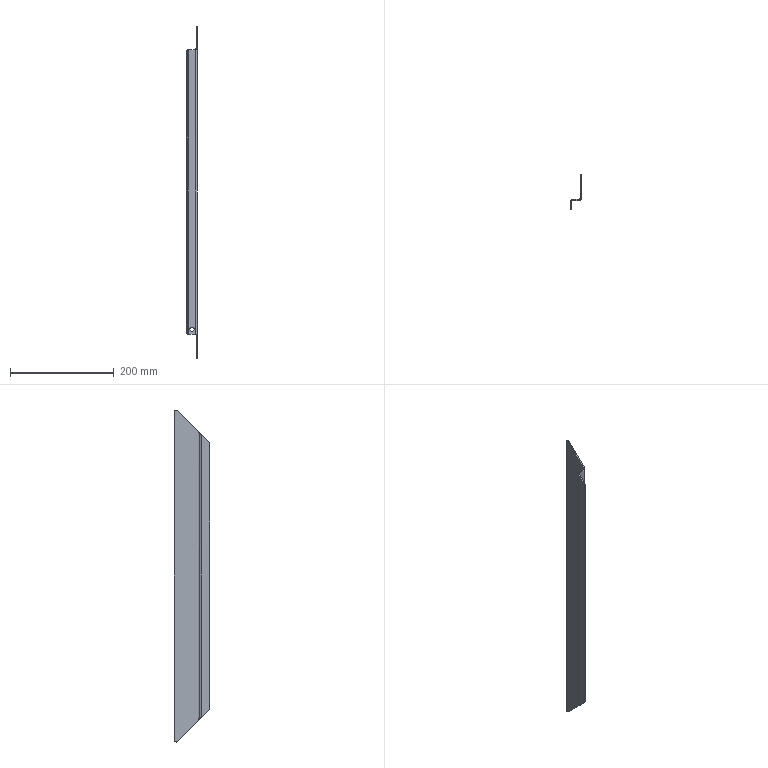Component | SolidWorks | BoxWelding-1_FrontAndRearPlate3-1 | 1 solid | 27 faces | box 20 x 68 x 641.51 mm | volume 95964 mm3 | plane 14 | cylinder 9 | spline 4 | commonest cylinder face diameters 8 x4 6 x3 4 x2
STEP:
#1=COLOUR_RGB('',0.7922,0.8196,0.9333);
#2=FILL_AREA_STYLE_COLOUR('',#1);
#3=FILL_AREA_STYLE('',(#2));
#4=SURFACE_STYLE_FILL_AREA(#3);
#5=SURFACE_SIDE_STYLE('',(#4));
#6=SURFACE_STYLE_USAGE(.BOTH.,#5);
#7=PRESENTATION_STYLE_ASSIGNMENT((#6));
#8=CARTESIAN_POINT('',(22.269,49.429,-6.496));
#9=VERTEX_POINT('',#8);
#10=CARTESIAN_POINT('',(21.954,49.429,-6.496));
#11=VERTEX_POINT('',#10);
#12=CARTESIAN_POINT('',(22.111,49.429,-6.496));
#13=DIRECTION('',(0.,-1.,0.));
#14=DIRECTION('',(-1.,0.,-0.));
#15=AXIS2_PLACEMENT_3D('',#12,#13,#14);
#16=CIRCLE('',#15,0.1575);
#17=EDGE_CURVE('',#9,#11,#16,.T.);
#18=ORIENTED_EDGE('',*,*,#17,.F.);
#19=CARTESIAN_POINT('',(22.269,49.35,-6.496));
#20=VERTEX_POINT('',#19);
#21=CARTESIAN_POINT('',(22.269,49.744,-6.496));
#22=DIRECTION('',(0.,-1.,0.));
#23=VECTOR('',#22,39.37);
#24=LINE('',#21,#23);
#25=EDGE_CURVE('',#9,#20,#24,.T.);
#26=ORIENTED_EDGE('',*,*,#25,.T.);
#27=CARTESIAN_POINT('',(21.954,49.35,-6.496));
#28=VERTEX_POINT('',#27);
#29=CARTESIAN_POINT('',(22.111,49.35,-6.496));
#30=DIRECTION('',(0.,-1.,0.));
#31=DIRECTION('',(-1.,0.,-0.));
#32=AXIS2_PLACEMENT_3D('',#29,#30,#31);
#33=CIRCLE('',#32,0.1575);
#34=EDGE_CURVE('',#20,#28,#33,.T.);
#35=ORIENTED_EDGE('',*,*,#34,.T.);
#36=CARTESIAN_POINT('',(21.954,49.744,-6.496));
#37=DIRECTION('',(0.,-1.,0.));
#38=VECTOR('',#37,39.37);
#39=LINE('',#36,#38);
#40=EDGE_CURVE('',#11,#28,#39,.T.);
#41=ORIENTED_EDGE('',*,*,#40,.F.);
#42=EDGE_LOOP('',(#18,#26,#35,#41));
#43=FACE_OUTER_BOUND('',#42,.T.);
#44=CARTESIAN_POINT('',(22.111,49.744,-6.496));
#45=DIRECTION('',(0.,-1.,0.));
#46=DIRECTION('',(-1.,0.,-0.));
#47=AXIS2_PLACEMENT_3D('',#44,#45,#46);
#48=CYLINDRICAL_SURFACE('',#47,0.1575);
#49=ADVANCED_FACE('',(#43),#48,.F.);
#50=CARTESIAN_POINT('',(22.505,51.201,16.566));
#51=VERTEX_POINT('',#50);
#52=CARTESIAN_POINT('',(22.505,51.117,16.531));
#53=VERTEX_POINT('',#52);
#54=CARTESIAN_POINT('',(22.505,51.201,16.448));
#55=DIRECTION('',(1.,0.,0.));
#56=DIRECTION('',(0.,-0.,-1.));
#57=AXIS2_PLACEMENT_3D('',#54,#55,#56);
#58=CIRCLE('',#57,0.1181);
#59=EDGE_CURVE('',#51,#53,#58,.T.);
#60=ORIENTED_EDGE('',*,*,#59,.F.);
#61=CARTESIAN_POINT('',(22.426,51.201,16.566));
#62=VERTEX_POINT('',#61);
#63=CARTESIAN_POINT('',(22.505,51.201,16.566));
#64=DIRECTION('',(-1.,-0.,-0.));
#65=VECTOR('',#64,39.37);
#66=LINE('',#63,#65);
#67=EDGE_CURVE('',#51,#62,#66,.T.);
#68=ORIENTED_EDGE('',*,*,#67,.T.);
#69=CARTESIAN_POINT('',(22.426,51.117,16.531));
#70=VERTEX_POINT('',#69);
#71=CARTESIAN_POINT('',(22.426,51.201,16.448));
#72=DIRECTION('',(-1.,-0.,-0.));
#73=DIRECTION('',(0.,-0.,-1.));
#74=AXIS2_PLACEMENT_3D('',#71,#72,#73);
#75=CIRCLE('',#74,0.1181);
#76=EDGE_CURVE('',#70,#62,#75,.T.);
#77=ORIENTED_EDGE('',*,*,#76,.F.);
#78=CARTESIAN_POINT('',(22.426,51.117,16.531));
#79=DIRECTION('',(-1.,-0.,-0.));
#80=VECTOR('',#79,39.37);
#81=LINE('',#78,#80);
#82=EDGE_CURVE('',#53,#70,#81,.T.);
#83=ORIENTED_EDGE('',*,*,#82,.F.);
#84=EDGE_LOOP('',(#60,#68,#77,#83));
#85=FACE_OUTER_BOUND('',#84,.T.);
#86=CARTESIAN_POINT('',(22.505,51.201,16.448));
#87=DIRECTION('',(-1.,-0.,-0.));
#88=DIRECTION('',(0.,0.,1.));
#89=AXIS2_PLACEMENT_3D('',#86,#87,#88);
#90=CYLINDRICAL_SURFACE('',#89,0.1181);
#91=ADVANCED_FACE('',(#85),#90,.T.);
#92=CARTESIAN_POINT('',(22.111,49.35,-6.496));
#93=DIRECTION('',(0.,-1.,0.));
#94=DIRECTION('',(-1.,0.,-0.));
#95=AXIS2_PLACEMENT_3D('',#92,#93,#94);
#96=CIRCLE('',#95,0.1575);
#97=EDGE_CURVE('',#28,#20,#96,.T.);
#98=ORIENTED_EDGE('',*,*,#97,.F.);
#99=ORIENTED_EDGE('',*,*,#34,.F.);
#100=EDGE_LOOP('',(#98,#99));
#101=FACE_BOUND('',#100,.T.);
#102=CARTESIAN_POINT('',(22.347,49.35,-6.889));
#103=VERTEX_POINT('',#102);
#104=CARTESIAN_POINT('',(22.347,49.35,14.764));
#105=VERTEX_POINT('',#104);
#106=CARTESIAN_POINT('',(22.347,49.35,16.733));
#107=DIRECTION('',(-0.,0.,1.));
#108=VECTOR('',#107,39.37);
#109=LINE('',#106,#108);
#110=EDGE_CURVE('',#103,#105,#109,.T.);
#111=ORIENTED_EDGE('',*,*,#110,.T.);
#112=CARTESIAN_POINT('',(21.875,49.35,14.764));
#113=VERTEX_POINT('',#112);
#114=CARTESIAN_POINT('',(22.426,49.35,14.764));
#115=DIRECTION('',(1.,0.,0.));
#116=VECTOR('',#115,39.37);
#117=LINE('',#114,#116);
#118=EDGE_CURVE('',#113,#105,#117,.T.);
#119=ORIENTED_EDGE('',*,*,#118,.F.);
#120=CARTESIAN_POINT('',(21.875,49.35,-6.889));
#121=VERTEX_POINT('',#120);
#122=CARTESIAN_POINT('',(21.875,49.35,-8.858));
#123=DIRECTION('',(-0.,0.,1.));
#124=VECTOR('',#123,39.37);
#125=LINE('',#122,#124);
#126=EDGE_CURVE('',#121,#113,#125,.T.);
#127=ORIENTED_EDGE('',*,*,#126,.F.);
#128=CARTESIAN_POINT('',(22.426,49.35,-6.889));
#129=DIRECTION('',(-1.,-0.,-0.));
#130=VECTOR('',#129,39.37);
#131=LINE('',#128,#130);
#132=EDGE_CURVE('',#103,#121,#131,.T.);
#133=ORIENTED_EDGE('',*,*,#132,.F.);
#134=EDGE_LOOP('',(#111,#119,#127,#133));
#135=FACE_OUTER_BOUND('',#134,.T.);
#136=CARTESIAN_POINT('',(22.426,49.35,16.733));
#137=DIRECTION('',(0.,-1.,0.));
#138=DIRECTION('',(-1.,-0.,-0.));
#139=AXIS2_PLACEMENT_3D('',#136,#137,#138);
#140=PLANE('',#139);
#141=ADVANCED_FACE('',(#101,#135),#140,.T.);
#142=CARTESIAN_POINT('',(22.111,49.429,-6.496));
#143=DIRECTION('',(0.,-1.,0.));
#144=DIRECTION('',(-1.,0.,-0.));
#145=AXIS2_PLACEMENT_3D('',#142,#143,#144);
#146=CIRCLE('',#145,0.1575);
#147=EDGE_CURVE('',#11,#9,#146,.T.);
#148=ORIENTED_EDGE('',*,*,#147,.T.);
#149=ORIENTED_EDGE('',*,*,#17,.T.);
#150=EDGE_LOOP('',(#148,#149));
#151=FACE_BOUND('',#150,.T.);
#152=CARTESIAN_POINT('',(21.875,49.429,14.764));
#153=VERTEX_POINT('',#152);
#154=CARTESIAN_POINT('',(22.347,49.429,14.764));
#155=VERTEX_POINT('',#154);
#156=CARTESIAN_POINT('',(22.426,49.429,14.764));
#157=DIRECTION('',(1.,0.,0.));
#158=VECTOR('',#157,39.37);
#159=LINE('',#156,#158);
#160=EDGE_CURVE('',#153,#155,#159,.T.);
#161=ORIENTED_EDGE('',*,*,#160,.T.);
#162=CARTESIAN_POINT('',(22.347,49.429,-6.889));
#163=VERTEX_POINT('',#162);
#164=CARTESIAN_POINT('',(22.347,49.429,-8.858));
#165=DIRECTION('',(-0.,0.,1.));
#166=VECTOR('',#165,39.37);
#167=LINE('',#164,#166);
#168=EDGE_CURVE('',#163,#155,#167,.T.);
#169=ORIENTED_EDGE('',*,*,#168,.F.);
#170=CARTESIAN_POINT('',(21.875,49.429,-6.889));
#171=VERTEX_POINT('',#170);
#172=CARTESIAN_POINT('',(22.426,49.429,-6.889));
#173=DIRECTION('',(-1.,-0.,-0.));
#174=VECTOR('',#173,39.37);
#175=LINE('',#172,#174);
#176=EDGE_CURVE('',#163,#171,#175,.T.);
#177=ORIENTED_EDGE('',*,*,#176,.T.);
#178=CARTESIAN_POINT('',(21.875,49.429,-8.858));
#179=DIRECTION('',(-0.,0.,1.));
#180=VECTOR('',#179,39.37);
#181=LINE('',#178,#180);
#182=EDGE_CURVE('',#171,#153,#181,.T.);
#183=ORIENTED_EDGE('',*,*,#182,.T.);
#184=EDGE_LOOP('',(#161,#169,#177,#183));
#185=FACE_OUTER_BOUND('',#184,.T.);
#186=CARTESIAN_POINT('',(22.426,49.429,16.733));
#187=DIRECTION('',(0.,-1.,0.));
#188=DIRECTION('',(-1.,-0.,-0.));
#189=AXIS2_PLACEMENT_3D('',#186,#187,#188);
#190=PLANE('',#189);
#191=ADVANCED_FACE('',(#151,#185),#190,.F.);
#192=CARTESIAN_POINT('',(22.505,51.319,-8.573));
#193=VERTEX_POINT('',#192);
#194=CARTESIAN_POINT('',(22.505,51.319,16.448));
#195=VERTEX_POINT('',#194);
#196=CARTESIAN_POINT('',(22.505,51.319,16.733));
#197=DIRECTION('',(-0.,0.,1.));
#198=VECTOR('',#197,39.37);
#199=LINE('',#196,#198);
#200=EDGE_CURVE('',#193,#195,#199,.T.);
#201=ORIENTED_EDGE('',*,*,#200,.T.);
#202=CARTESIAN_POINT('',(22.505,51.201,16.448));
#203=DIRECTION('',(1.,0.,0.));
#204=DIRECTION('',(0.,-0.,-1.));
#205=AXIS2_PLACEMENT_3D('',#202,#203,#204);
#206=CIRCLE('',#205,0.1181);
#207=EDGE_CURVE('',#195,#51,#206,.T.);
#208=ORIENTED_EDGE('',*,*,#207,.T.);
#209=ORIENTED_EDGE('',*,*,#59,.T.);
#210=CARTESIAN_POINT('',(22.505,49.508,14.922));
#211=VERTEX_POINT('',#210);
#212=CARTESIAN_POINT('',(22.505,37.539,2.953));
#213=DIRECTION('',(-0.,0.7071,0.7071));
#214=VECTOR('',#213,39.37);
#215=LINE('',#212,#214);
#216=EDGE_CURVE('',#211,#53,#215,.T.);
#217=ORIENTED_EDGE('',*,*,#216,.F.);
#218=CARTESIAN_POINT('',(22.505,49.508,-7.047));
#219=VERTEX_POINT('',#218);
#220=CARTESIAN_POINT('',(22.505,49.508,16.733));
#221=DIRECTION('',(0.,-0.,-1.));
#222=VECTOR('',#221,39.37);
#223=LINE('',#220,#222);
#224=EDGE_CURVE('',#211,#219,#223,.T.);
#225=ORIENTED_EDGE('',*,*,#224,.T.);
#226=CARTESIAN_POINT('',(22.505,51.117,-8.656));
#227=VERTEX_POINT('',#226);
#228=CARTESIAN_POINT('',(22.505,50.335,-7.874));
#229=DIRECTION('',(0.,-0.7071,0.7071));
#230=VECTOR('',#229,39.37);
#231=LINE('',#228,#230);
#232=EDGE_CURVE('',#227,#219,#231,.T.);
#233=ORIENTED_EDGE('',*,*,#232,.F.);
#234=CARTESIAN_POINT('',(22.505,51.201,-8.573));
#235=DIRECTION('',(1.,0.,0.));
#236=DIRECTION('',(0.,-0.,-1.));
#237=AXIS2_PLACEMENT_3D('',#234,#235,#236);
#238=CIRCLE('',#237,0.1181);
#239=EDGE_CURVE('',#227,#193,#238,.T.);
#240=ORIENTED_EDGE('',*,*,#239,.T.);
#241=EDGE_LOOP('',(#201,#208,#209,#217,#225,#233,#240));
#242=FACE_OUTER_BOUND('',#241,.T.);
#243=CARTESIAN_POINT('',(22.505,49.35,-8.858));
#244=DIRECTION('',(1.,0.,0.));
#245=DIRECTION('',(0.,-0.,-1.));
#246=AXIS2_PLACEMENT_3D('',#243,#244,#245);
#247=PLANE('',#246);
#248=ADVANCED_FACE('',(#242),#247,.T.);
#249=CARTESIAN_POINT('',(22.426,49.508,14.922));
#250=VERTEX_POINT('',#249);
#251=CARTESIAN_POINT('',(22.426,37.539,2.953));
#252=DIRECTION('',(-0.,0.7071,0.7071));
#253=VECTOR('',#252,39.37);
#254=LINE('',#251,#253);
#255=EDGE_CURVE('',#250,#70,#254,.T.);
#256=ORIENTED_EDGE('',*,*,#255,.T.);
#257=ORIENTED_EDGE('',*,*,#76,.T.);
#258=CARTESIAN_POINT('',(22.426,51.319,16.448));
#259=VERTEX_POINT('',#258);
#260=CARTESIAN_POINT('',(22.426,51.201,16.448));
#261=DIRECTION('',(-1.,-0.,-0.));
#262=DIRECTION('',(0.,-0.,-1.));
#263=AXIS2_PLACEMENT_3D('',#260,#261,#262);
#264=CIRCLE('',#263,0.1181);
#265=EDGE_CURVE('',#62,#259,#264,.T.);
#266=ORIENTED_EDGE('',*,*,#265,.T.);
#267=CARTESIAN_POINT('',(22.426,51.319,-8.573));
#268=VERTEX_POINT('',#267);
#269=CARTESIAN_POINT('',(22.426,51.319,-8.858));
#270=DIRECTION('',(-0.,0.,1.));
#271=VECTOR('',#270,39.37);
#272=LINE('',#269,#271);
#273=EDGE_CURVE('',#268,#259,#272,.T.);
#274=ORIENTED_EDGE('',*,*,#273,.F.);
#275=CARTESIAN_POINT('',(22.426,51.117,-8.656));
#276=VERTEX_POINT('',#275);
#277=CARTESIAN_POINT('',(22.426,51.201,-8.573));
#278=DIRECTION('',(-1.,-0.,-0.));
#279=DIRECTION('',(0.,-0.,-1.));
#280=AXIS2_PLACEMENT_3D('',#277,#278,#279);
#281=CIRCLE('',#280,0.1181);
#282=EDGE_CURVE('',#268,#276,#281,.T.);
#283=ORIENTED_EDGE('',*,*,#282,.T.);
#284=CARTESIAN_POINT('',(22.426,49.508,-7.047));
#285=VERTEX_POINT('',#284);
#286=CARTESIAN_POINT('',(22.426,50.335,-7.874));
#287=DIRECTION('',(0.,-0.7071,0.7071));
#288=VECTOR('',#287,39.37);
#289=LINE('',#286,#288);
#290=EDGE_CURVE('',#276,#285,#289,.T.);
#291=ORIENTED_EDGE('',*,*,#290,.T.);
#292=CARTESIAN_POINT('',(22.426,49.508,16.733));
#293=DIRECTION('',(0.,-0.,-1.));
#294=VECTOR('',#293,39.37);
#295=LINE('',#292,#294);
#296=EDGE_CURVE('',#250,#285,#295,.T.);
#297=ORIENTED_EDGE('',*,*,#296,.F.);
#298=EDGE_LOOP('',(#256,#257,#266,#274,#283,#291,#297));
#299=FACE_OUTER_BOUND('',#298,.T.);
#300=CARTESIAN_POINT('',(22.426,49.35,-8.858));
#301=DIRECTION('',(1.,0.,0.));
#302=DIRECTION('',(0.,-0.,-1.));
#303=AXIS2_PLACEMENT_3D('',#300,#301,#302);
#304=PLANE('',#303);
#305=ADVANCED_FACE('',(#299),#304,.F.);
#306=ORIENTED_EDGE('',*,*,#224,.F.);
#307=CARTESIAN_POINT('',(22.347,49.35,14.764));
#308=CARTESIAN_POINT('',(22.44,49.35,14.764));
#309=CARTESIAN_POINT('',(22.505,49.416,14.83));
#310=CARTESIAN_POINT('',(22.505,49.508,14.922));
#311=(BOUNDED_CURVE()B_SPLINE_CURVE(3,(#307,#308,#309,#310),.UNSPECIFIED.,.F.,.T.)B_SPLINE_CURVE_WITH_KNOTS((4,4),(3.142,4.712),.UNSPECIFIED.)CURVE()GEOMETRIC_REPRESENTATION_ITEM()RATIONAL_B_SPLINE_CURVE((1.,0.8047,0.8047,1.))REPRESENTATION_ITEM(''));
#312=EDGE_CURVE('',#105,#211,#311,.T.);
#313=ORIENTED_EDGE('',*,*,#312,.F.);
#314=ORIENTED_EDGE('',*,*,#110,.F.);
#315=CARTESIAN_POINT('',(22.505,49.508,-7.047));
#316=CARTESIAN_POINT('',(22.505,49.416,-6.954));
#317=CARTESIAN_POINT('',(22.44,49.35,-6.889));
#318=CARTESIAN_POINT('',(22.347,49.35,-6.889));
#319=(BOUNDED_CURVE()B_SPLINE_CURVE(3,(#315,#316,#317,#318),.UNSPECIFIED.,.F.,.F.)B_SPLINE_CURVE_WITH_KNOTS((4,4),(4.712,6.283),.UNSPECIFIED.)CURVE()GEOMETRIC_REPRESENTATION_ITEM()RATIONAL_B_SPLINE_CURVE((1.,0.8047,0.8047,1.))REPRESENTATION_ITEM(''));
#320=EDGE_CURVE('',#219,#103,#319,.T.);
#321=ORIENTED_EDGE('',*,*,#320,.F.);
#322=EDGE_LOOP('',(#306,#313,#314,#321));
#323=FACE_OUTER_BOUND('',#322,.T.);
#324=CARTESIAN_POINT('',(22.347,49.508,16.733));
#325=DIRECTION('',(-0.,0.,1.));
#326=DIRECTION('',(0.,-1.,0.));
#327=AXIS2_PLACEMENT_3D('',#324,#325,#326);
#328=CYLINDRICAL_SURFACE('',#327,0.1575);
#329=ADVANCED_FACE('',(#323),#328,.T.);
#330=CARTESIAN_POINT('',(22.347,49.429,14.764));
#331=CARTESIAN_POINT('',(22.393,49.429,14.764));
#332=CARTESIAN_POINT('',(22.426,49.462,14.83));
#333=CARTESIAN_POINT('',(22.426,49.508,14.922));
#334=(BOUNDED_CURVE()B_SPLINE_CURVE(3,(#330,#331,#332,#333),.UNSPECIFIED.,.F.,.F.)B_SPLINE_CURVE_WITH_KNOTS((4,4),(3.142,4.712),.UNSPECIFIED.)CURVE()GEOMETRIC_REPRESENTATION_ITEM()RATIONAL_B_SPLINE_CURVE((1.,0.8047,0.8047,1.))REPRESENTATION_ITEM(''));
#335=EDGE_CURVE('',#155,#250,#334,.T.);
#336=ORIENTED_EDGE('',*,*,#335,.T.);
#337=ORIENTED_EDGE('',*,*,#296,.T.);
#338=CARTESIAN_POINT('',(22.426,49.508,-7.047));
#339=CARTESIAN_POINT('',(22.426,49.462,-6.954));
#340=CARTESIAN_POINT('',(22.393,49.429,-6.889));
#341=CARTESIAN_POINT('',(22.347,49.429,-6.889));
#342=(BOUNDED_CURVE()B_SPLINE_CURVE(3,(#338,#339,#340,#341),.UNSPECIFIED.,.F.,.F.)B_SPLINE_CURVE_WITH_KNOTS((4,4),(4.712,6.283),.UNSPECIFIED.)CURVE()GEOMETRIC_REPRESENTATION_ITEM()RATIONAL_B_SPLINE_CURVE((1.,0.8047,0.8047,1.))REPRESENTATION_ITEM(''));
#343=EDGE_CURVE('',#285,#163,#342,.T.);
#344=ORIENTED_EDGE('',*,*,#343,.T.);
#345=ORIENTED_EDGE('',*,*,#168,.T.);
#346=EDGE_LOOP('',(#336,#337,#344,#345));
#347=FACE_OUTER_BOUND('',#346,.T.);
#348=CARTESIAN_POINT('',(22.347,49.508,16.733));
#349=DIRECTION('',(-0.,0.,1.));
#350=DIRECTION('',(0.,-1.,0.));
#351=AXIS2_PLACEMENT_3D('',#348,#349,#350);
#352=CYLINDRICAL_SURFACE('',#351,0.07874);
#353=ADVANCED_FACE('',(#347),#352,.F.);
#354=CARTESIAN_POINT('',(21.717,49.272,14.686));
#355=VERTEX_POINT('',#354);
#356=CARTESIAN_POINT('',(21.717,49.272,-6.811));
#357=VERTEX_POINT('',#356);
#358=CARTESIAN_POINT('',(21.717,49.272,-8.858));
#359=DIRECTION('',(0.,-0.,-1.));
#360=VECTOR('',#359,39.37);
#361=LINE('',#358,#360);
#362=EDGE_CURVE('',#355,#357,#361,.T.);
#363=ORIENTED_EDGE('',*,*,#362,.F.);
#364=CARTESIAN_POINT('',(21.875,49.429,14.764));
#365=CARTESIAN_POINT('',(21.783,49.429,14.764));
#366=CARTESIAN_POINT('',(21.717,49.364,14.732));
#367=CARTESIAN_POINT('',(21.717,49.272,14.686));
#368=(BOUNDED_CURVE()B_SPLINE_CURVE(3,(#364,#365,#366,#367),.UNSPECIFIED.,.F.,.T.)B_SPLINE_CURVE_WITH_KNOTS((4,4),(3.142,4.712),.UNSPECIFIED.)CURVE()GEOMETRIC_REPRESENTATION_ITEM()RATIONAL_B_SPLINE_CURVE((1.,0.8047,0.8047,1.))REPRESENTATION_ITEM(''));
#369=EDGE_CURVE('',#153,#355,#368,.T.);
#370=ORIENTED_EDGE('',*,*,#369,.F.);
#371=ORIENTED_EDGE('',*,*,#182,.F.);
#372=CARTESIAN_POINT('',(21.717,49.272,-6.811));
#373=CARTESIAN_POINT('',(21.717,49.364,-6.857));
#374=CARTESIAN_POINT('',(21.783,49.429,-6.889));
#375=CARTESIAN_POINT('',(21.875,49.429,-6.889));
#376=(BOUNDED_CURVE()B_SPLINE_CURVE(3,(#372,#373,#374,#375),.UNSPECIFIED.,.F.,.T.)B_SPLINE_CURVE_WITH_KNOTS((4,4),(4.712,6.283),.UNSPECIFIED.)CURVE()GEOMETRIC_REPRESENTATION_ITEM()RATIONAL_B_SPLINE_CURVE((1.,0.8047,0.8047,1.))REPRESENTATION_ITEM(''));
#377=EDGE_CURVE('',#357,#171,#376,.T.);
#378=ORIENTED_EDGE('',*,*,#377,.F.);
#379=EDGE_LOOP('',(#363,#370,#371,#378));
#380=FACE_OUTER_BOUND('',#379,.T.);
#381=CARTESIAN_POINT('',(21.875,49.272,-8.858));
#382=DIRECTION('',(0.,-0.,-1.));
#383=DIRECTION('',(-1.,0.,-0.));
#384=AXIS2_PLACEMENT_3D('',#381,#382,#383);
#385=CYLINDRICAL_SURFACE('',#384,0.1575);
#386=ADVANCED_FACE('',(#380),#385,.T.);
#387=CARTESIAN_POINT('',(21.796,49.272,14.686));
#388=VERTEX_POINT('',#387);
#389=CARTESIAN_POINT('',(21.875,49.35,14.764));
#390=CARTESIAN_POINT('',(21.829,49.35,14.764));
#391=CARTESIAN_POINT('',(21.796,49.318,14.732));
#392=CARTESIAN_POINT('',(21.796,49.272,14.686));
#393=(BOUNDED_CURVE()B_SPLINE_CURVE(3,(#389,#390,#391,#392),.UNSPECIFIED.,.F.,.F.)B_SPLINE_CURVE_WITH_KNOTS((4,4),(3.142,4.712),.UNSPECIFIED.)CURVE()GEOMETRIC_REPRESENTATION_ITEM()RATIONAL_B_SPLINE_CURVE((1.,0.8047,0.8047,1.))REPRESENTATION_ITEM(''));
#394=EDGE_CURVE('',#113,#388,#393,.T.);
#395=ORIENTED_EDGE('',*,*,#394,.T.);
#396=CARTESIAN_POINT('',(21.796,49.272,-6.811));
#397=VERTEX_POINT('',#396);
#398=CARTESIAN_POINT('',(21.796,49.272,16.733));
#399=DIRECTION('',(0.,-0.,-1.));
#400=VECTOR('',#399,39.37);
#401=LINE('',#398,#400);
#402=EDGE_CURVE('',#388,#397,#401,.T.);
#403=ORIENTED_EDGE('',*,*,#402,.T.);
#404=CARTESIAN_POINT('',(21.796,49.272,-6.811));
#405=CARTESIAN_POINT('',(21.796,49.318,-6.857));
#406=CARTESIAN_POINT('',(21.829,49.35,-6.889));
#407=CARTESIAN_POINT('',(21.875,49.35,-6.889));
#408=(BOUNDED_CURVE()B_SPLINE_CURVE(3,(#404,#405,#406,#407),.UNSPECIFIED.,.F.,.F.)B_SPLINE_CURVE_WITH_KNOTS((4,4),(4.712,6.283),.UNSPECIFIED.)CURVE()GEOMETRIC_REPRESENTATION_ITEM()RATIONAL_B_SPLINE_CURVE((1.,0.8047,0.8047,1.))REPRESENTATION_ITEM(''));
#409=EDGE_CURVE('',#397,#121,#408,.T.);
#410=ORIENTED_EDGE('',*,*,#409,.T.);
#411=ORIENTED_EDGE('',*,*,#126,.T.);
#412=EDGE_LOOP('',(#395,#403,#410,#411));
#413=FACE_OUTER_BOUND('',#412,.T.);
#414=CARTESIAN_POINT('',(21.875,49.272,-8.858));
#415=DIRECTION('',(0.,-0.,-1.));
#416=DIRECTION('',(-1.,0.,0.));
#417=AXIS2_PLACEMENT_3D('',#414,#415,#416);
#418=CYLINDRICAL_SURFACE('',#417,0.07874);
#419=ADVANCED_FACE('',(#413),#418,.F.);
#420=CARTESIAN_POINT('',(21.717,48.642,14.056));
#421=VERTEX_POINT('',#420);
#422=CARTESIAN_POINT('',(21.717,48.642,-6.181));
#423=VERTEX_POINT('',#422);
#424=CARTESIAN_POINT('',(21.717,48.642,-8.858));
#425=DIRECTION('',(0.,-0.,-1.));
#426=VECTOR('',#425,39.37);
#427=LINE('',#424,#426);
#428=EDGE_CURVE('',#421,#423,#427,.T.);
#429=ORIENTED_EDGE('',*,*,#428,.F.);
#430=CARTESIAN_POINT('',(21.717,37.539,2.953));
#431=DIRECTION('',(0.,-0.7071,-0.7071));
#432=VECTOR('',#431,39.37);
#433=LINE('',#430,#432);
#434=EDGE_CURVE('',#355,#421,#433,.T.);
#435=ORIENTED_EDGE('',*,*,#434,.F.);
#436=ORIENTED_EDGE('',*,*,#362,.T.);
#437=CARTESIAN_POINT('',(21.717,51.319,-8.858));
#438=DIRECTION('',(0.,-0.7071,0.7071));
#439=VECTOR('',#438,39.37);
#440=LINE('',#437,#439);
#441=EDGE_CURVE('',#357,#423,#440,.T.);
#442=ORIENTED_EDGE('',*,*,#441,.T.);
#443=EDGE_LOOP('',(#429,#435,#436,#442));
#444=FACE_OUTER_BOUND('',#443,.T.);
#445=CARTESIAN_POINT('',(21.717,49.35,-8.858));
#446=DIRECTION('',(-1.,-0.,-0.));
#447=DIRECTION('',(-0.,0.,1.));
#448=AXIS2_PLACEMENT_3D('',#445,#446,#447);
#449=PLANE('',#448);
#450=ADVANCED_FACE('',(#444),#449,.T.);
#451=CARTESIAN_POINT('',(21.796,48.642,14.056));
#452=VERTEX_POINT('',#451);
#453=CARTESIAN_POINT('',(21.796,37.539,2.953));
#454=DIRECTION('',(0.,-0.7071,-0.7071));
#455=VECTOR('',#454,39.37);
#456=LINE('',#453,#455);
#457=EDGE_CURVE('',#388,#452,#456,.T.);
#458=ORIENTED_EDGE('',*,*,#457,.T.);
#459=CARTESIAN_POINT('',(21.796,48.642,-6.181));
#460=VERTEX_POINT('',#459);
#461=CARTESIAN_POINT('',(21.796,48.642,-8.858));
#462=DIRECTION('',(0.,-0.,-1.));
#463=VECTOR('',#462,39.37);
#464=LINE('',#461,#463);
#465=EDGE_CURVE('',#452,#460,#464,.T.);
#466=ORIENTED_EDGE('',*,*,#465,.T.);
#467=CARTESIAN_POINT('',(21.796,51.319,-8.858));
#468=DIRECTION('',(0.,-0.7071,0.7071));
#469=VECTOR('',#468,39.37);
#470=LINE('',#467,#469);
#471=EDGE_CURVE('',#397,#460,#470,.T.);
#472=ORIENTED_EDGE('',*,*,#471,.F.);
#473=ORIENTED_EDGE('',*,*,#402,.F.);
#474=EDGE_LOOP('',(#458,#466,#472,#473));
#475=FACE_OUTER_BOUND('',#474,.T.);
#476=CARTESIAN_POINT('',(21.796,49.35,-8.858));
#477=DIRECTION('',(-1.,-0.,-0.));
#478=DIRECTION('',(-0.,0.,1.));
#479=AXIS2_PLACEMENT_3D('',#476,#477,#478);
#480=PLANE('',#479);
#481=ADVANCED_FACE('',(#475),#480,.F.);
#482=ORIENTED_EDGE('',*,*,#465,.F.);
#483=CARTESIAN_POINT('',(21.796,48.642,14.056));
#484=DIRECTION('',(-1.,-0.,-0.));
#485=VECTOR('',#484,39.37);
#486=LINE('',#483,#485);
#487=EDGE_CURVE('',#452,#421,#486,.T.);
#488=ORIENTED_EDGE('',*,*,#487,.T.);
#489=ORIENTED_EDGE('',*,*,#428,.T.);
#490=CARTESIAN_POINT('',(21.717,48.642,-6.181));
#491=DIRECTION('',(1.,0.,0.));
#492=VECTOR('',#491,39.37);
#493=LINE('',#490,#492);
#494=EDGE_CURVE('',#423,#460,#493,.T.);
#495=ORIENTED_EDGE('',*,*,#494,.T.);
#496=EDGE_LOOP('',(#482,#488,#489,#495));
#497=FACE_OUTER_BOUND('',#496,.T.);
#498=CARTESIAN_POINT('',(21.717,48.642,-8.858));
#499=DIRECTION('',(0.,-1.,0.));
#500=DIRECTION('',(-1.,-0.,-0.));
#501=AXIS2_PLACEMENT_3D('',#498,#499,#500);
#502=PLANE('',#501);
#503=ADVANCED_FACE('',(#497),#502,.T.);
#504=ORIENTED_EDGE('',*,*,#273,.T.);
#505=CARTESIAN_POINT('',(22.505,51.319,16.448));
#506=DIRECTION('',(1.,0.,0.));
#507=VECTOR('',#506,39.37);
#508=LINE('',#505,#507);
#509=EDGE_CURVE('',#259,#195,#508,.T.);
#510=ORIENTED_EDGE('',*,*,#509,.T.);
#511=ORIENTED_EDGE('',*,*,#200,.F.);
#512=CARTESIAN_POINT('',(22.505,51.319,-8.573));
#513=DIRECTION('',(-1.,-0.,-0.));
#514=VECTOR('',#513,39.37);
#515=LINE('',#512,#514);
#516=EDGE_CURVE('',#193,#268,#515,.T.);
#517=ORIENTED_EDGE('',*,*,#516,.T.);
#518=EDGE_LOOP('',(#504,#510,#511,#517));
#519=FACE_OUTER_BOUND('',#518,.T.);
#520=CARTESIAN_POINT('',(22.505,51.319,16.733));
#521=DIRECTION('',(-0.,1.,-0.));
#522=DIRECTION('',(-0.,0.,1.));
#523=AXIS2_PLACEMENT_3D('',#520,#521,#522);
#524=PLANE('',#523);
#525=ADVANCED_FACE('',(#519),#524,.T.);
#526=ORIENTED_EDGE('',*,*,#290,.F.);
#527=CARTESIAN_POINT('',(22.426,51.117,-8.656));
#528=DIRECTION('',(1.,0.,0.));
#529=VECTOR('',#528,39.37);
#530=LINE('',#527,#529);
#531=EDGE_CURVE('',#276,#227,#530,.T.);
#532=ORIENTED_EDGE('',*,*,#531,.T.);
#533=ORIENTED_EDGE('',*,*,#232,.T.);
#534=CARTESIAN_POINT('',(22.426,49.508,-7.047));
#535=DIRECTION('',(1.,0.,0.));
#536=VECTOR('',#535,39.37);
#537=LINE('',#534,#536);
#538=EDGE_CURVE('',#285,#219,#537,.T.);
#539=ORIENTED_EDGE('',*,*,#538,.F.);
#540=EDGE_LOOP('',(#526,#532,#533,#539));
#541=FACE_OUTER_BOUND('',#540,.T.);
#542=CARTESIAN_POINT('',(22.426,50.335,-7.874));
#543=DIRECTION('',(-0.,0.7071,0.7071));
#544=DIRECTION('',(0.,-0.7071,0.7071));
#545=AXIS2_PLACEMENT_3D('',#542,#543,#544);
#546=PLANE('',#545);
#547=ADVANCED_FACE('',(#541),#546,.F.);
#548=ORIENTED_EDGE('',*,*,#132,.T.);
#549=CARTESIAN_POINT('',(21.875,49.35,-6.889));
#550=DIRECTION('',(-0.,1.,-0.));
#551=VECTOR('',#550,39.37);
#552=LINE('',#549,#551);
#553=EDGE_CURVE('',#121,#171,#552,.T.);
#554=ORIENTED_EDGE('',*,*,#553,.T.);
#555=ORIENTED_EDGE('',*,*,#176,.F.);
#556=CARTESIAN_POINT('',(22.347,49.35,-6.889));
#557=DIRECTION('',(-0.,1.,-0.));
#558=VECTOR('',#557,39.37);
#559=LINE('',#556,#558);
#560=EDGE_CURVE('',#103,#163,#559,.T.);
#561=ORIENTED_EDGE('',*,*,#560,.F.);
#562=EDGE_LOOP('',(#548,#554,#555,#561));
#563=FACE_OUTER_BOUND('',#562,.T.);
#564=CARTESIAN_POINT('',(22.426,49.35,-6.889));
#565=DIRECTION('',(-0.,0.,1.));
#566=DIRECTION('',(-1.,-0.,-0.));
#567=AXIS2_PLACEMENT_3D('',#564,#565,#566);
#568=PLANE('',#567);
#569=ADVANCED_FACE('',(#563),#568,.F.);
#570=ORIENTED_EDGE('',*,*,#441,.F.);
#571=CARTESIAN_POINT('',(21.717,49.272,-6.811));
#572=DIRECTION('',(1.,0.,0.));
#573=VECTOR('',#572,39.37);
#574=LINE('',#571,#573);
#575=EDGE_CURVE('',#357,#397,#574,.T.);
#576=ORIENTED_EDGE('',*,*,#575,.T.);
#577=ORIENTED_EDGE('',*,*,#471,.T.);
#578=ORIENTED_EDGE('',*,*,#494,.F.);
#579=EDGE_LOOP('',(#570,#576,#577,#578));
#580=FACE_OUTER_BOUND('',#579,.T.);
#581=CARTESIAN_POINT('',(21.717,51.319,-8.858));
#582=DIRECTION('',(0.,-0.7071,-0.7071));
#583=DIRECTION('',(0.,-0.7071,0.7071));
#584=AXIS2_PLACEMENT_3D('',#581,#582,#583);
#585=PLANE('',#584);
#586=ADVANCED_FACE('',(#580),#585,.T.);
#587=ORIENTED_EDGE('',*,*,#553,.F.);
#588=ORIENTED_EDGE('',*,*,#409,.F.);
#589=ORIENTED_EDGE('',*,*,#575,.F.);
#590=ORIENTED_EDGE('',*,*,#377,.T.);
#591=EDGE_LOOP('',(#587,#588,#589,#590));
#592=FACE_OUTER_BOUND('',#591,.T.);
#593=CARTESIAN_POINT('',(21.875,49.429,-6.889));
#594=CARTESIAN_POINT('',(21.875,49.403,-6.889));
#595=CARTESIAN_POINT('',(21.875,49.377,-6.889));
#596=CARTESIAN_POINT('',(21.875,49.35,-6.889));
#597=CARTESIAN_POINT('',(22.19,49.429,-6.889));
#598=CARTESIAN_POINT('',(22.137,49.403,-6.889));
#599=CARTESIAN_POINT('',(22.085,49.377,-6.889));
#600=CARTESIAN_POINT('',(22.032,49.35,-6.889));
#601=CARTESIAN_POINT('',(22.19,49.114,-6.732));
#602=CARTESIAN_POINT('',(22.137,49.14,-6.732));
#603=CARTESIAN_POINT('',(22.085,49.167,-6.732));
#604=CARTESIAN_POINT('',(22.032,49.193,-6.732));
#605=CARTESIAN_POINT('',(21.875,49.114,-6.732));
#606=CARTESIAN_POINT('',(21.875,49.14,-6.732));
#607=CARTESIAN_POINT('',(21.875,49.167,-6.732));
#608=CARTESIAN_POINT('',(21.875,49.193,-6.732));
#609=CARTESIAN_POINT('',(21.56,49.114,-6.732));
#610=CARTESIAN_POINT('',(21.612,49.14,-6.732));
#611=CARTESIAN_POINT('',(21.665,49.167,-6.732));
#612=CARTESIAN_POINT('',(21.717,49.193,-6.732));
#613=CARTESIAN_POINT('',(21.56,49.429,-6.889));
#614=CARTESIAN_POINT('',(21.612,49.403,-6.889));
#615=CARTESIAN_POINT('',(21.665,49.377,-6.889));
#616=CARTESIAN_POINT('',(21.717,49.35,-6.889));
#617=CARTESIAN_POINT('',(21.875,49.429,-6.889));
#618=CARTESIAN_POINT('',(21.875,49.403,-6.889));
#619=CARTESIAN_POINT('',(21.875,49.377,-6.889));
#620=CARTESIAN_POINT('',(21.875,49.35,-6.889));
#621=(BOUNDED_SURFACE()B_SPLINE_SURFACE(3,3,((#593,#594,#595,#596),(#597,#598,#599,#600),(#601,#602,#603,#604),(#605,#606,#607,#608),(#609,#610,#611,#612),(#613,#614,#615,#616),(#617,#618,#619,#620)),.UNSPECIFIED.,.T.,.F.,.F.)B_SPLINE_SURFACE_WITH_KNOTS((4,3,4),(4,4),(0.,0.5,1.),(0.,1.),.UNSPECIFIED.)GEOMETRIC_REPRESENTATION_ITEM()RATIONAL_B_SPLINE_SURFACE(((1.,1.,1.,1.),(0.3333,0.3333,0.3333,0.3333),(0.3333,0.3333,0.3333,0.3333),(1.,1.,1.,1.),(0.3333,0.3333,0.3333,0.3333),(0.3333,0.3333,0.3333,0.3333),(1.,1.,1.,1.)))REPRESENTATION_ITEM('')SURFACE());
#622=ADVANCED_FACE('',(#592),#621,.T.);
#623=ORIENTED_EDGE('',*,*,#320,.T.);
#624=ORIENTED_EDGE('',*,*,#560,.T.);
#625=ORIENTED_EDGE('',*,*,#343,.F.);
#626=ORIENTED_EDGE('',*,*,#538,.T.);
#627=EDGE_LOOP('',(#623,#624,#625,#626));
#628=FACE_OUTER_BOUND('',#627,.T.);
#629=CARTESIAN_POINT('',(22.347,49.35,-6.889));
#630=CARTESIAN_POINT('',(22.347,49.377,-6.889));
#631=CARTESIAN_POINT('',(22.347,49.403,-6.889));
#632=CARTESIAN_POINT('',(22.347,49.429,-6.889));
#633=CARTESIAN_POINT('',(22.032,49.35,-6.889));
#634=CARTESIAN_POINT('',(22.085,49.377,-6.889));
#635=CARTESIAN_POINT('',(22.137,49.403,-6.889));
#636=CARTESIAN_POINT('',(22.19,49.429,-6.889));
#637=CARTESIAN_POINT('',(22.032,49.665,-7.204));
#638=CARTESIAN_POINT('',(22.085,49.639,-7.204));
#639=CARTESIAN_POINT('',(22.137,49.613,-7.204));
#640=CARTESIAN_POINT('',(22.19,49.587,-7.204));
#641=CARTESIAN_POINT('',(22.347,49.665,-7.204));
#642=CARTESIAN_POINT('',(22.347,49.639,-7.204));
#643=CARTESIAN_POINT('',(22.347,49.613,-7.204));
#644=CARTESIAN_POINT('',(22.347,49.587,-7.204));
#645=CARTESIAN_POINT('',(22.662,49.665,-7.204));
#646=CARTESIAN_POINT('',(22.61,49.639,-7.204));
#647=CARTESIAN_POINT('',(22.557,49.613,-7.204));
#648=CARTESIAN_POINT('',(22.505,49.587,-7.204));
#649=CARTESIAN_POINT('',(22.662,49.35,-6.889));
#650=CARTESIAN_POINT('',(22.61,49.377,-6.889));
#651=CARTESIAN_POINT('',(22.557,49.403,-6.889));
#652=CARTESIAN_POINT('',(22.505,49.429,-6.889));
#653=CARTESIAN_POINT('',(22.347,49.35,-6.889));
#654=CARTESIAN_POINT('',(22.347,49.377,-6.889));
#655=CARTESIAN_POINT('',(22.347,49.403,-6.889));
#656=CARTESIAN_POINT('',(22.347,49.429,-6.889));
#657=(BOUNDED_SURFACE()B_SPLINE_SURFACE(3,3,((#629,#630,#631,#632),(#633,#634,#635,#636),(#637,#638,#639,#640),(#641,#642,#643,#644),(#645,#646,#647,#648),(#649,#650,#651,#652),(#653,#654,#655,#656)),.UNSPECIFIED.,.T.,.F.,.F.)B_SPLINE_SURFACE_WITH_KNOTS((4,3,4),(4,4),(0.,0.5,1.),(0.,1.),.UNSPECIFIED.)GEOMETRIC_REPRESENTATION_ITEM()RATIONAL_B_SPLINE_SURFACE(((1.,1.,1.,1.),(0.3333,0.3333,0.3333,0.3333),(0.3333,0.3333,0.3333,0.3333),(1.,1.,1.,1.),(0.3333,0.3333,0.3333,0.3333),(0.3333,0.3333,0.3333,0.3333),(1.,1.,1.,1.)))REPRESENTATION_ITEM('')SURFACE());
#658=ADVANCED_FACE('',(#628),#657,.T.);
#659=ORIENTED_EDGE('',*,*,#216,.T.);
#660=ORIENTED_EDGE('',*,*,#82,.T.);
#661=ORIENTED_EDGE('',*,*,#255,.F.);
#662=CARTESIAN_POINT('',(22.426,49.508,14.922));
#663=DIRECTION('',(1.,0.,0.));
#664=VECTOR('',#663,39.37);
#665=LINE('',#662,#664);
#666=EDGE_CURVE('',#250,#211,#665,.T.);
#667=ORIENTED_EDGE('',*,*,#666,.T.);
#668=EDGE_LOOP('',(#659,#660,#661,#667));
#669=FACE_OUTER_BOUND('',#668,.T.);
#670=CARTESIAN_POINT('',(22.426,37.539,2.953));
#671=DIRECTION('',(-0.,0.7071,-0.7071));
#672=DIRECTION('',(-0.,0.7071,0.7071));
#673=AXIS2_PLACEMENT_3D('',#670,#671,#672);
#674=PLANE('',#673);
#675=ADVANCED_FACE('',(#669),#674,.F.);
#676=ORIENTED_EDGE('',*,*,#118,.T.);
#677=CARTESIAN_POINT('',(22.347,49.35,14.764));
#678=DIRECTION('',(-0.,1.,-0.));
#679=VECTOR('',#678,39.37);
#680=LINE('',#677,#679);
#681=EDGE_CURVE('',#105,#155,#680,.T.);
#682=ORIENTED_EDGE('',*,*,#681,.T.);
#683=ORIENTED_EDGE('',*,*,#160,.F.);
#684=CARTESIAN_POINT('',(21.875,49.35,14.764));
#685=DIRECTION('',(-0.,1.,-0.));
#686=VECTOR('',#685,39.37);
#687=LINE('',#684,#686);
#688=EDGE_CURVE('',#113,#153,#687,.T.);
#689=ORIENTED_EDGE('',*,*,#688,.F.);
#690=EDGE_LOOP('',(#676,#682,#683,#689));
#691=FACE_OUTER_BOUND('',#690,.T.);
#692=CARTESIAN_POINT('',(22.426,49.35,14.764));
#693=DIRECTION('',(0.,-0.,-1.));
#694=DIRECTION('',(1.,0.,0.));
#695=AXIS2_PLACEMENT_3D('',#692,#693,#694);
#696=PLANE('',#695);
#697=ADVANCED_FACE('',(#691),#696,.F.);
#698=ORIENTED_EDGE('',*,*,#487,.F.);
#699=ORIENTED_EDGE('',*,*,#457,.F.);
#700=CARTESIAN_POINT('',(21.796,49.272,14.686));
#701=DIRECTION('',(-1.,-0.,-0.));
#702=VECTOR('',#701,39.37);
#703=LINE('',#700,#702);
#704=EDGE_CURVE('',#388,#355,#703,.T.);
#705=ORIENTED_EDGE('',*,*,#704,.T.);
#706=ORIENTED_EDGE('',*,*,#434,.T.);
#707=EDGE_LOOP('',(#698,#699,#705,#706));
#708=FACE_OUTER_BOUND('',#707,.T.);
#709=CARTESIAN_POINT('',(21.796,37.539,2.953));
#710=DIRECTION('',(-0.,0.7071,-0.7071));
#711=DIRECTION('',(0.,-0.7071,-0.7071));
#712=AXIS2_PLACEMENT_3D('',#709,#710,#711);
#713=PLANE('',#712);
#714=ADVANCED_FACE('',(#708),#713,.F.);
#715=ORIENTED_EDGE('',*,*,#704,.F.);
#716=ORIENTED_EDGE('',*,*,#394,.F.);
#717=ORIENTED_EDGE('',*,*,#688,.T.);
#718=ORIENTED_EDGE('',*,*,#369,.T.);
#719=EDGE_LOOP('',(#715,#716,#717,#718));
#720=FACE_OUTER_BOUND('',#719,.T.);
#721=CARTESIAN_POINT('',(21.875,49.114,14.607));
#722=CARTESIAN_POINT('',(21.875,49.14,14.607));
#723=CARTESIAN_POINT('',(21.875,49.167,14.607));
#724=CARTESIAN_POINT('',(21.875,49.193,14.607));
#725=CARTESIAN_POINT('',(22.19,49.114,14.607));
#726=CARTESIAN_POINT('',(22.137,49.14,14.607));
#727=CARTESIAN_POINT('',(22.085,49.167,14.607));
#728=CARTESIAN_POINT('',(22.032,49.193,14.607));
#729=CARTESIAN_POINT('',(22.19,49.429,14.764));
#730=CARTESIAN_POINT('',(22.137,49.403,14.764));
#731=CARTESIAN_POINT('',(22.085,49.377,14.764));
#732=CARTESIAN_POINT('',(22.032,49.35,14.764));
#733=CARTESIAN_POINT('',(21.875,49.429,14.764));
#734=CARTESIAN_POINT('',(21.875,49.403,14.764));
#735=CARTESIAN_POINT('',(21.875,49.377,14.764));
#736=CARTESIAN_POINT('',(21.875,49.35,14.764));
#737=CARTESIAN_POINT('',(21.56,49.429,14.764));
#738=CARTESIAN_POINT('',(21.612,49.403,14.764));
#739=CARTESIAN_POINT('',(21.665,49.377,14.764));
#740=CARTESIAN_POINT('',(21.717,49.35,14.764));
#741=CARTESIAN_POINT('',(21.56,49.114,14.607));
#742=CARTESIAN_POINT('',(21.612,49.14,14.607));
#743=CARTESIAN_POINT('',(21.665,49.167,14.607));
#744=CARTESIAN_POINT('',(21.717,49.193,14.607));
#745=CARTESIAN_POINT('',(21.875,49.114,14.607));
#746=CARTESIAN_POINT('',(21.875,49.14,14.607));
#747=CARTESIAN_POINT('',(21.875,49.167,14.607));
#748=CARTESIAN_POINT('',(21.875,49.193,14.607));
#749=(BOUNDED_SURFACE()B_SPLINE_SURFACE(3,3,((#721,#722,#723,#724),(#725,#726,#727,#728),(#729,#730,#731,#732),(#733,#734,#735,#736),(#737,#738,#739,#740),(#741,#742,#743,#744),(#745,#746,#747,#748)),.UNSPECIFIED.,.T.,.F.,.F.)B_SPLINE_SURFACE_WITH_KNOTS((4,3,4),(4,4),(0.,0.5,1.),(0.,1.),.UNSPECIFIED.)GEOMETRIC_REPRESENTATION_ITEM()RATIONAL_B_SPLINE_SURFACE(((1.,1.,1.,1.),(0.3333,0.3333,0.3333,0.3333),(0.3333,0.3333,0.3333,0.3333),(1.,1.,1.,1.),(0.3333,0.3333,0.3333,0.3333),(0.3333,0.3333,0.3333,0.3333),(1.,1.,1.,1.)))REPRESENTATION_ITEM('')SURFACE());
#750=ADVANCED_FACE('',(#720),#749,.T.);
#751=ORIENTED_EDGE('',*,*,#312,.T.);
#752=ORIENTED_EDGE('',*,*,#666,.F.);
#753=ORIENTED_EDGE('',*,*,#335,.F.);
#754=ORIENTED_EDGE('',*,*,#681,.F.);
#755=EDGE_LOOP('',(#751,#752,#753,#754));
#756=FACE_OUTER_BOUND('',#755,.T.);
#757=CARTESIAN_POINT('',(22.347,49.665,15.079));
#758=CARTESIAN_POINT('',(22.347,49.639,15.079));
#759=CARTESIAN_POINT('',(22.347,49.613,15.079));
#760=CARTESIAN_POINT('',(22.347,49.587,15.079));
#761=CARTESIAN_POINT('',(22.032,49.665,15.079));
#762=CARTESIAN_POINT('',(22.085,49.639,15.079));
#763=CARTESIAN_POINT('',(22.137,49.613,15.079));
#764=CARTESIAN_POINT('',(22.19,49.587,15.079));
#765=CARTESIAN_POINT('',(22.032,49.35,14.764));
#766=CARTESIAN_POINT('',(22.085,49.377,14.764));
#767=CARTESIAN_POINT('',(22.137,49.403,14.764));
#768=CARTESIAN_POINT('',(22.19,49.429,14.764));
#769=CARTESIAN_POINT('',(22.347,49.35,14.764));
#770=CARTESIAN_POINT('',(22.347,49.377,14.764));
#771=CARTESIAN_POINT('',(22.347,49.403,14.764));
#772=CARTESIAN_POINT('',(22.347,49.429,14.764));
#773=CARTESIAN_POINT('',(22.662,49.35,14.764));
#774=CARTESIAN_POINT('',(22.61,49.377,14.764));
#775=CARTESIAN_POINT('',(22.557,49.403,14.764));
#776=CARTESIAN_POINT('',(22.505,49.429,14.764));
#777=CARTESIAN_POINT('',(22.662,49.665,15.079));
#778=CARTESIAN_POINT('',(22.61,49.639,15.079));
#779=CARTESIAN_POINT('',(22.557,49.613,15.079));
#780=CARTESIAN_POINT('',(22.505,49.587,15.079));
#781=CARTESIAN_POINT('',(22.347,49.665,15.079));
#782=CARTESIAN_POINT('',(22.347,49.639,15.079));
#783=CARTESIAN_POINT('',(22.347,49.613,15.079));
#784=CARTESIAN_POINT('',(22.347,49.587,15.079));
#785=(BOUNDED_SURFACE()B_SPLINE_SURFACE(3,3,((#757,#758,#759,#760),(#761,#762,#763,#764),(#765,#766,#767,#768),(#769,#770,#771,#772),(#773,#774,#775,#776),(#777,#778,#779,#780),(#781,#782,#783,#784)),.UNSPECIFIED.,.T.,.F.,.F.)B_SPLINE_SURFACE_WITH_KNOTS((4,3,4),(4,4),(0.,0.5,1.),(0.,1.),.UNSPECIFIED.)GEOMETRIC_REPRESENTATION_ITEM()RATIONAL_B_SPLINE_SURFACE(((1.,1.,1.,1.),(0.3333,0.3333,0.3333,0.3333),(0.3333,0.3333,0.3333,0.3333),(1.,1.,1.,1.),(0.3333,0.3333,0.3333,0.3333),(0.3333,0.3333,0.3333,0.3333),(1.,1.,1.,1.)))REPRESENTATION_ITEM('')SURFACE());
#786=ADVANCED_FACE('',(#756),#785,.T.);
#787=ORIENTED_EDGE('',*,*,#67,.F.);
#788=ORIENTED_EDGE('',*,*,#207,.F.);
#789=ORIENTED_EDGE('',*,*,#509,.F.);
#790=ORIENTED_EDGE('',*,*,#265,.F.);
#791=EDGE_LOOP('',(#787,#788,#789,#790));
#792=FACE_OUTER_BOUND('',#791,.T.);
#793=CARTESIAN_POINT('',(22.505,51.201,16.448));
#794=DIRECTION('',(-1.,-0.,-0.));
#795=DIRECTION('',(0.,0.,1.));
#796=AXIS2_PLACEMENT_3D('',#793,#794,#795);
#797=CYLINDRICAL_SURFACE('',#796,0.1181);
#798=ADVANCED_FACE('',(#792),#797,.T.);
#799=ORIENTED_EDGE('',*,*,#282,.F.);
#800=ORIENTED_EDGE('',*,*,#516,.F.);
#801=ORIENTED_EDGE('',*,*,#239,.F.);
#802=ORIENTED_EDGE('',*,*,#531,.F.);
#803=EDGE_LOOP('',(#799,#800,#801,#802));
#804=FACE_OUTER_BOUND('',#803,.T.);
#805=CARTESIAN_POINT('',(22.426,51.201,-8.573));
#806=DIRECTION('',(-1.,-0.,-0.));
#807=DIRECTION('',(0.,0.,1.));
#808=AXIS2_PLACEMENT_3D('',#805,#806,#807);
#809=CYLINDRICAL_SURFACE('',#808,0.1181);
#810=ADVANCED_FACE('',(#804),#809,.T.);
#811=ORIENTED_EDGE('',*,*,#25,.F.);
#812=ORIENTED_EDGE('',*,*,#147,.F.);
#813=ORIENTED_EDGE('',*,*,#40,.T.);
#814=ORIENTED_EDGE('',*,*,#97,.T.);
#815=EDGE_LOOP('',(#811,#812,#813,#814));
#816=FACE_OUTER_BOUND('',#815,.T.);
#817=CARTESIAN_POINT('',(22.111,49.744,-6.496));
#818=DIRECTION('',(0.,-1.,0.));
#819=DIRECTION('',(-1.,0.,-0.));
#820=AXIS2_PLACEMENT_3D('',#817,#818,#819);
#821=CYLINDRICAL_SURFACE('',#820,0.1575);
#822=ADVANCED_FACE('',(#816),#821,.F.);
#823=CLOSED_SHELL('',(#49,#91,#141,#191,#248,#305,#329,#353,#386,#419,#450,#481,#503,#525,#547,#569,#586,#622,#658,#675,#697,#714,#750,#786,#798,#810,#822));
#824=MANIFOLD_SOLID_BREP('',#823);
#825=STYLED_ITEM('',(#7),#824);
#826=(LENGTH_UNIT()NAMED_UNIT(*)SI_UNIT($,.METRE.));
#827=LENGTH_MEASURE_WITH_UNIT(LENGTH_MEASURE(0.0254),#826);
#828=DIMENSIONAL_EXPONENTS(1.,0.,0.,0.,0.,0.,0.);
#829=(CONVERSION_BASED_UNIT('',#827)LENGTH_UNIT()NAMED_UNIT(#828));
#830=UNCERTAINTY_MEASURE_WITH_UNIT(LENGTH_MEASURE(0.00001),#829,'','');
#831=(NAMED_UNIT(*)PLANE_ANGLE_UNIT()SI_UNIT($,.RADIAN.));
#832=(NAMED_UNIT(*)SI_UNIT($,.STERADIAN.)SOLID_ANGLE_UNIT());
#833=(GEOMETRIC_REPRESENTATION_CONTEXT(3)GLOBAL_UNCERTAINTY_ASSIGNED_CONTEXT((#830))GLOBAL_UNIT_ASSIGNED_CONTEXT((#829,#831,#832))REPRESENTATION_CONTEXT('',''));
#834=MECHANICAL_DESIGN_GEOMETRIC_PRESENTATION_REPRESENTATION('',(#825),#833);
#835=CARTESIAN_POINT('',(0.,0.,0.));
#836=DIRECTION('',(0.,0.,1.));
#837=DIRECTION('',(1.,0.,0.));
#838=AXIS2_PLACEMENT_3D('',#835,#836,#837);
#839=(LENGTH_UNIT()NAMED_UNIT(*)SI_UNIT($,.METRE.));
#840=LENGTH_MEASURE_WITH_UNIT(LENGTH_MEASURE(0.0254),#839);
#841=DIMENSIONAL_EXPONENTS(1.,0.,0.,0.,0.,0.,0.);
#842=(CONVERSION_BASED_UNIT('',#840)LENGTH_UNIT()NAMED_UNIT(#841));
#843=UNCERTAINTY_MEASURE_WITH_UNIT(LENGTH_MEASURE(0.00001),#842,'','');
#844=(NAMED_UNIT(*)PLANE_ANGLE_UNIT()SI_UNIT($,.RADIAN.));
#845=(NAMED_UNIT(*)SI_UNIT($,.STERADIAN.)SOLID_ANGLE_UNIT());
#846=(GEOMETRIC_REPRESENTATION_CONTEXT(3)GLOBAL_UNCERTAINTY_ASSIGNED_CONTEXT((#843))GLOBAL_UNIT_ASSIGNED_CONTEXT((#842,#844,#845))REPRESENTATION_CONTEXT('',''));
#847=ADVANCED_BREP_SHAPE_REPRESENTATION('',(#824,#838),#846);
#848=PRESENTATION_LAYER_ASSIGNMENT('','',(#825));